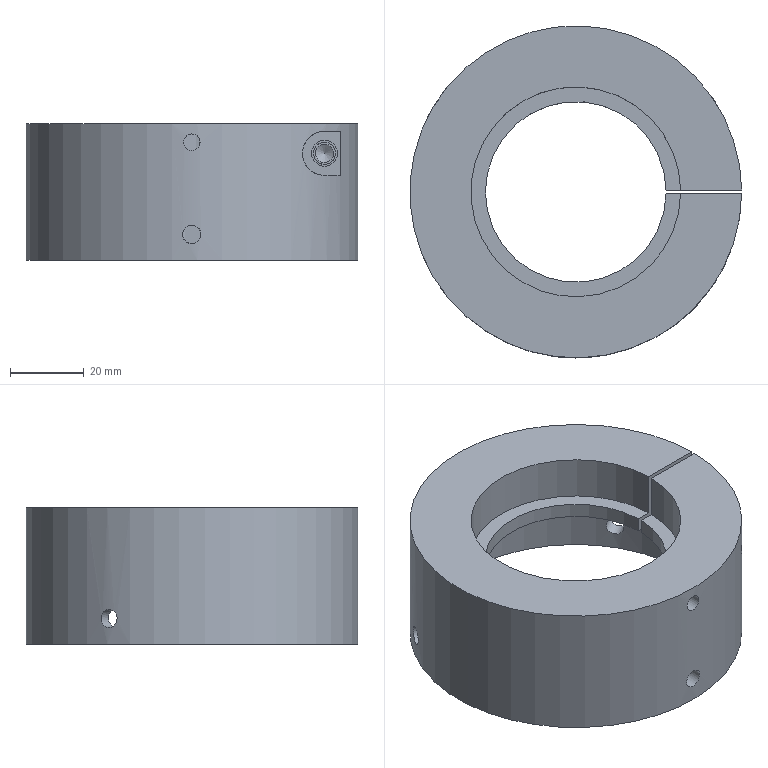Component | NX | CH3404_1-5 | 1 solid | 22 faces | volume 83702 mm3 | cylinder 11 | plane 10 | cone 1 | commonest cylinder face diameters 5 x3 90 x1 82 x1 49 x1 56.9 x1 4.5 x1 12 x1 7 x1